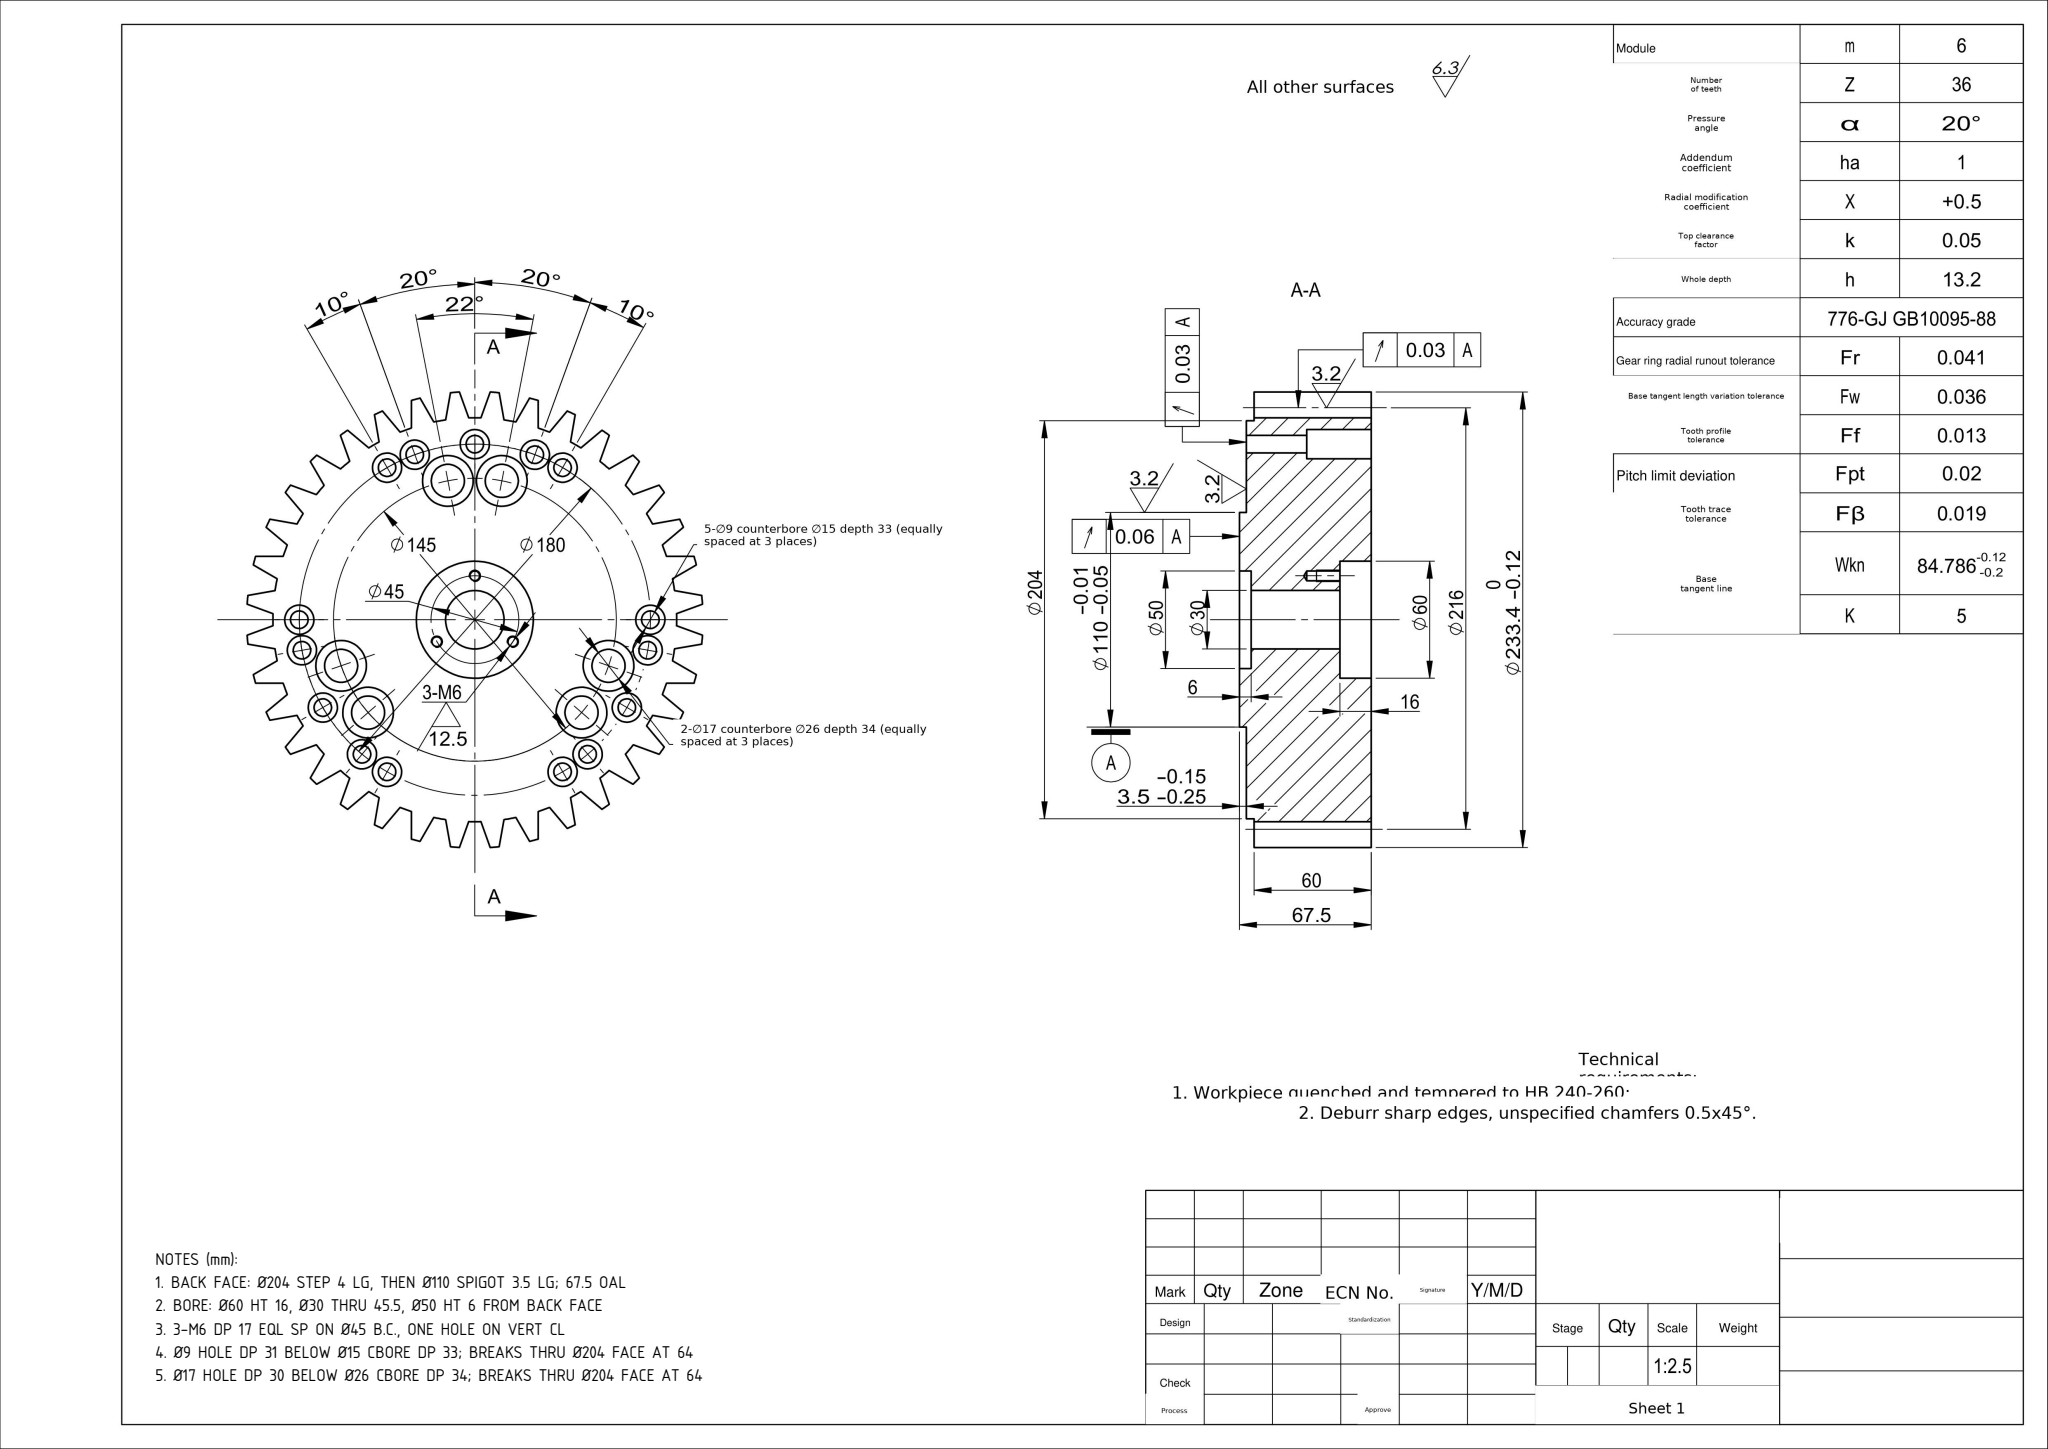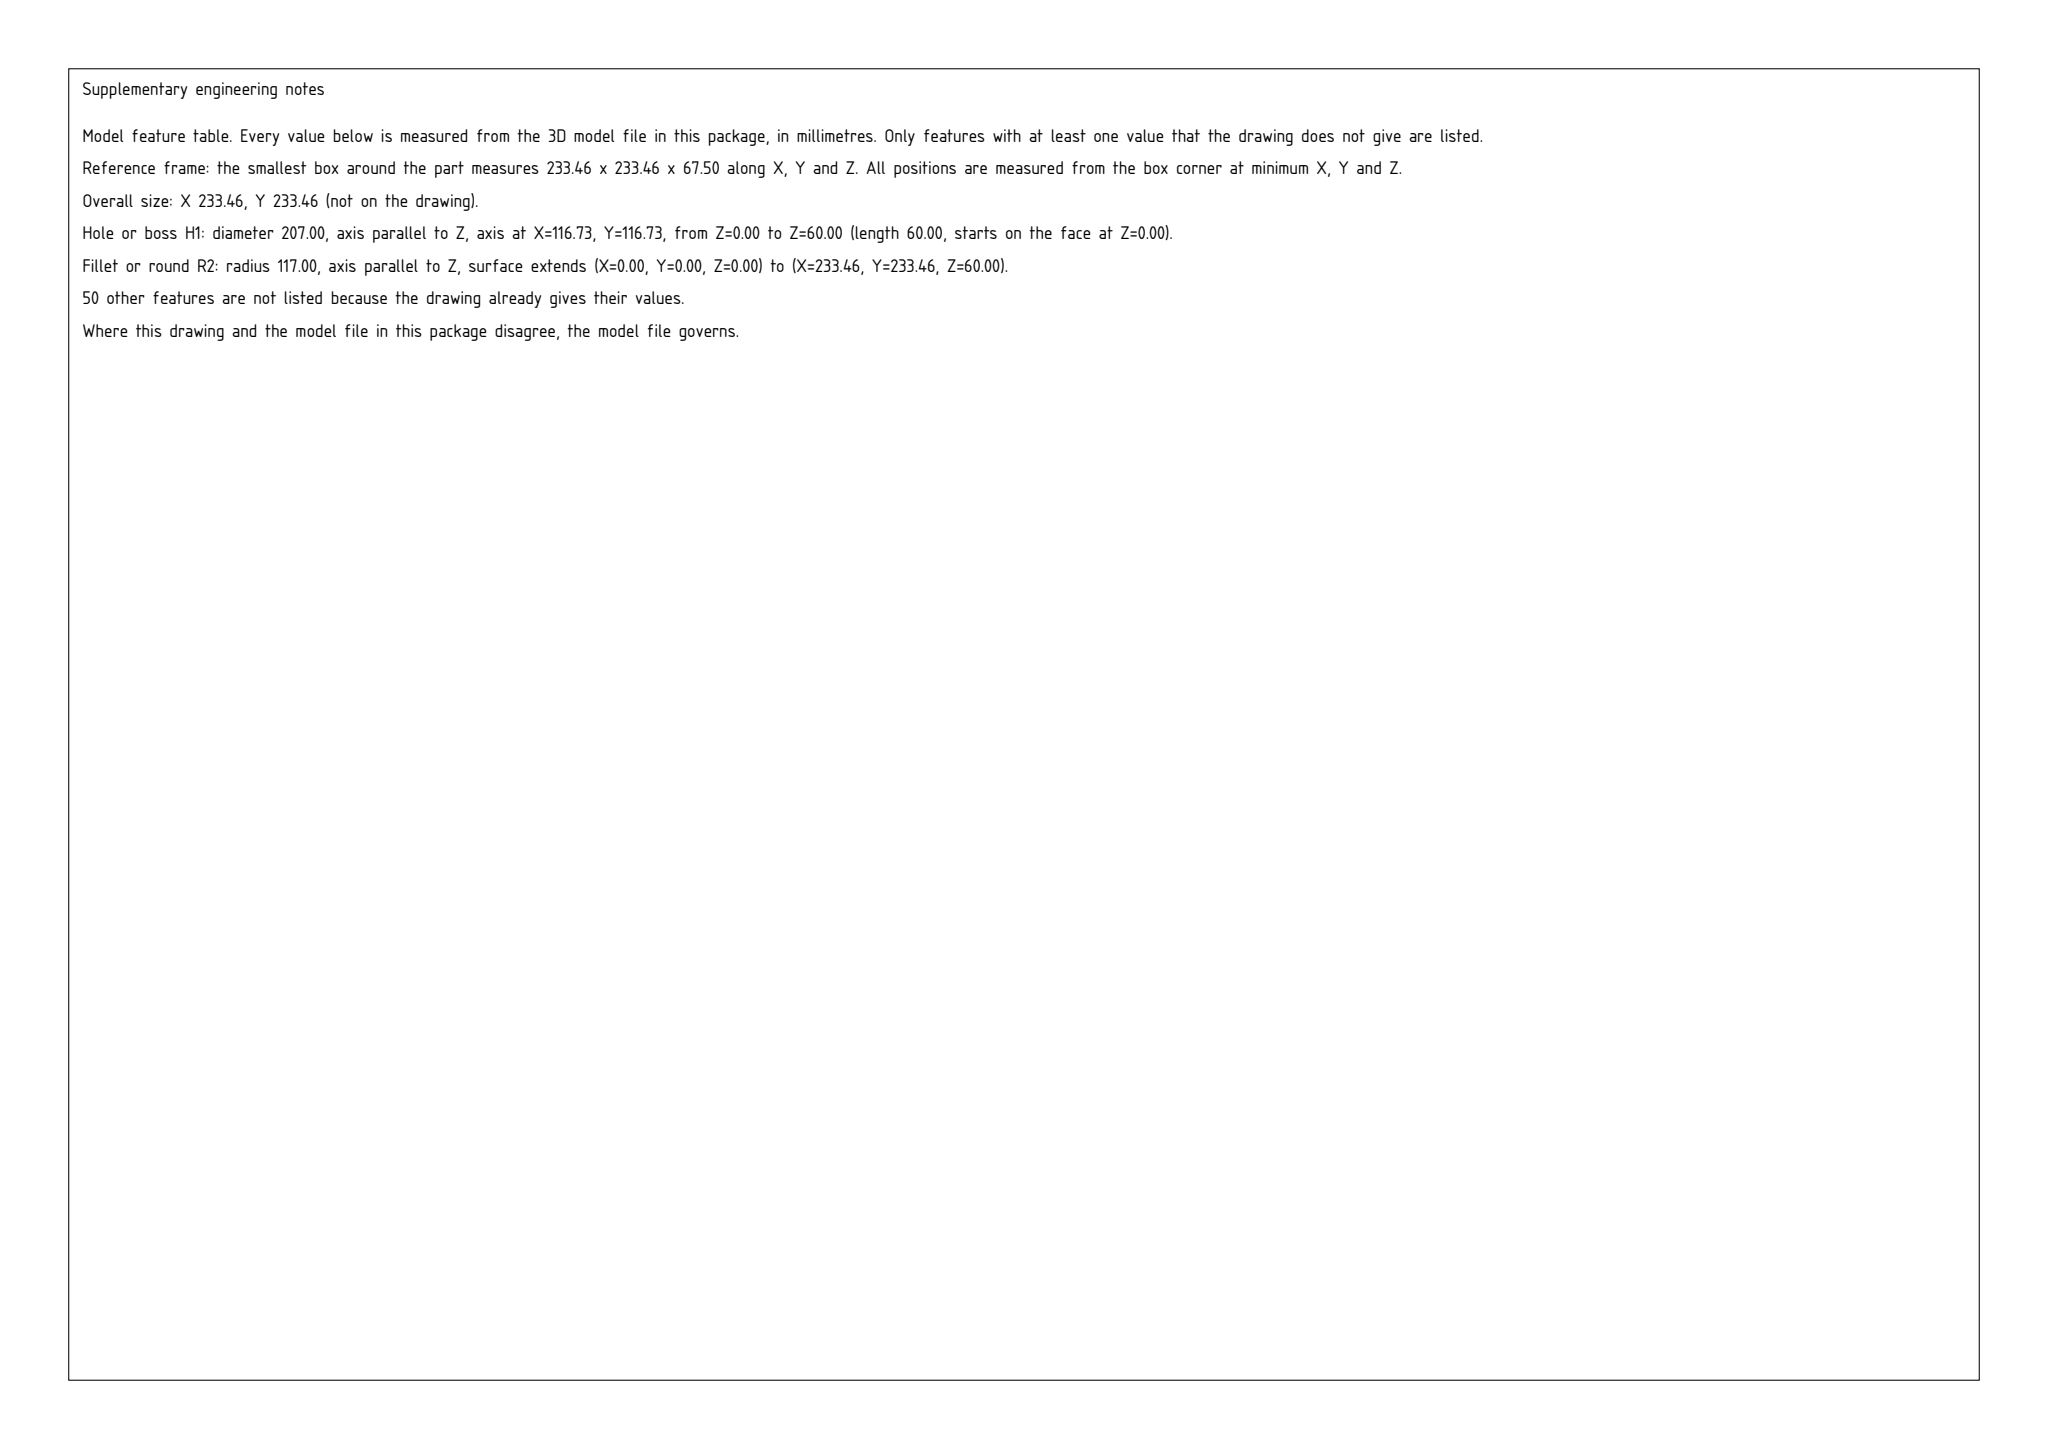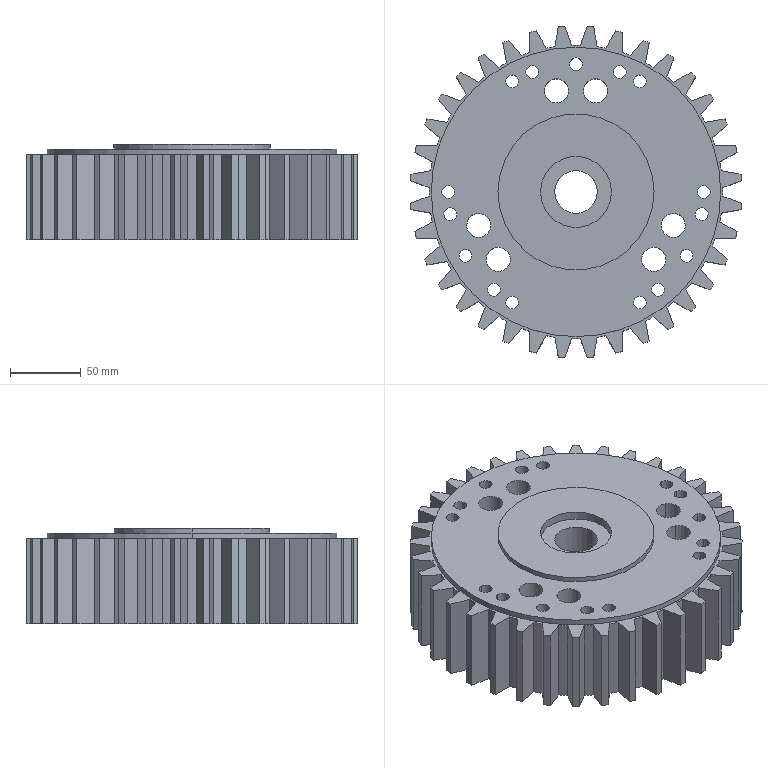Part | SolidWorks | mm | 1 solid | 277 faces | box 233.46 x 233.46 x 67.5 mm | volume 2066030 mm3 | cylinder 172 | plane 99 | cone 6 | commonest cylinder face diameters 234 x36 207 x36 15 x30 9 x30 26 x12 17 x12 5 x6 50 x2
Drawing notes:
BACK FACE: Ø204 STEP 4 LG, THEN Ø110 SPIGOT 3.5 LG; 67.5 OAL | from the solid: Ø204 z-cyl L=4.0 and Ø110 z-cyl L=3.5 on axis (116.73,116.73); z-planes 60, 64, 67.5 vs gear rim Ø234/Ø207 L=60; bbox z=67.5
BORE: Ø60 HT 16, Ø30 THRU 45.5, Ø50 HT 6 FROM BACK FACE | from the solid: Ø60 L=16 (z0-16), Ø30 L=45.5 (z16-61.5), Ø50 L=6 (z61.5-67.5), all on axis (116.73,116.73)
3-M6 DP 17 EQL SP ON Ø45 B.C., ONE HOLE ON VERT CL | from the solid: 3x Ø5.0 z-cyls L=17 at (97.25,105.48),(116.73,139.23),(136.22,105.48); R=22.5 from bore axis => Ø45 B.C. at 90/210/330°; 118° drill cone ref Ø5
Ø9 HOLE DP 31 BELOW Ø15 CBORE DP 33; BREAKS THRU Ø204 FACE AT 64 | from the solid: Ø9 cyl len 31 from z=33 to z=64; Ø15 cbore len 33 from z=0; z-plane 64 = Ø204 back-step face
Ø17 HOLE DP 30 BELOW Ø26 CBORE DP 34; BREAKS THRU Ø204 FACE AT 64 | from the solid: Ø17 cyl len 30 from z=34 to z=64; Ø26 cbore len 34 from z=0; z-plane 64 = Ø204 back-step face